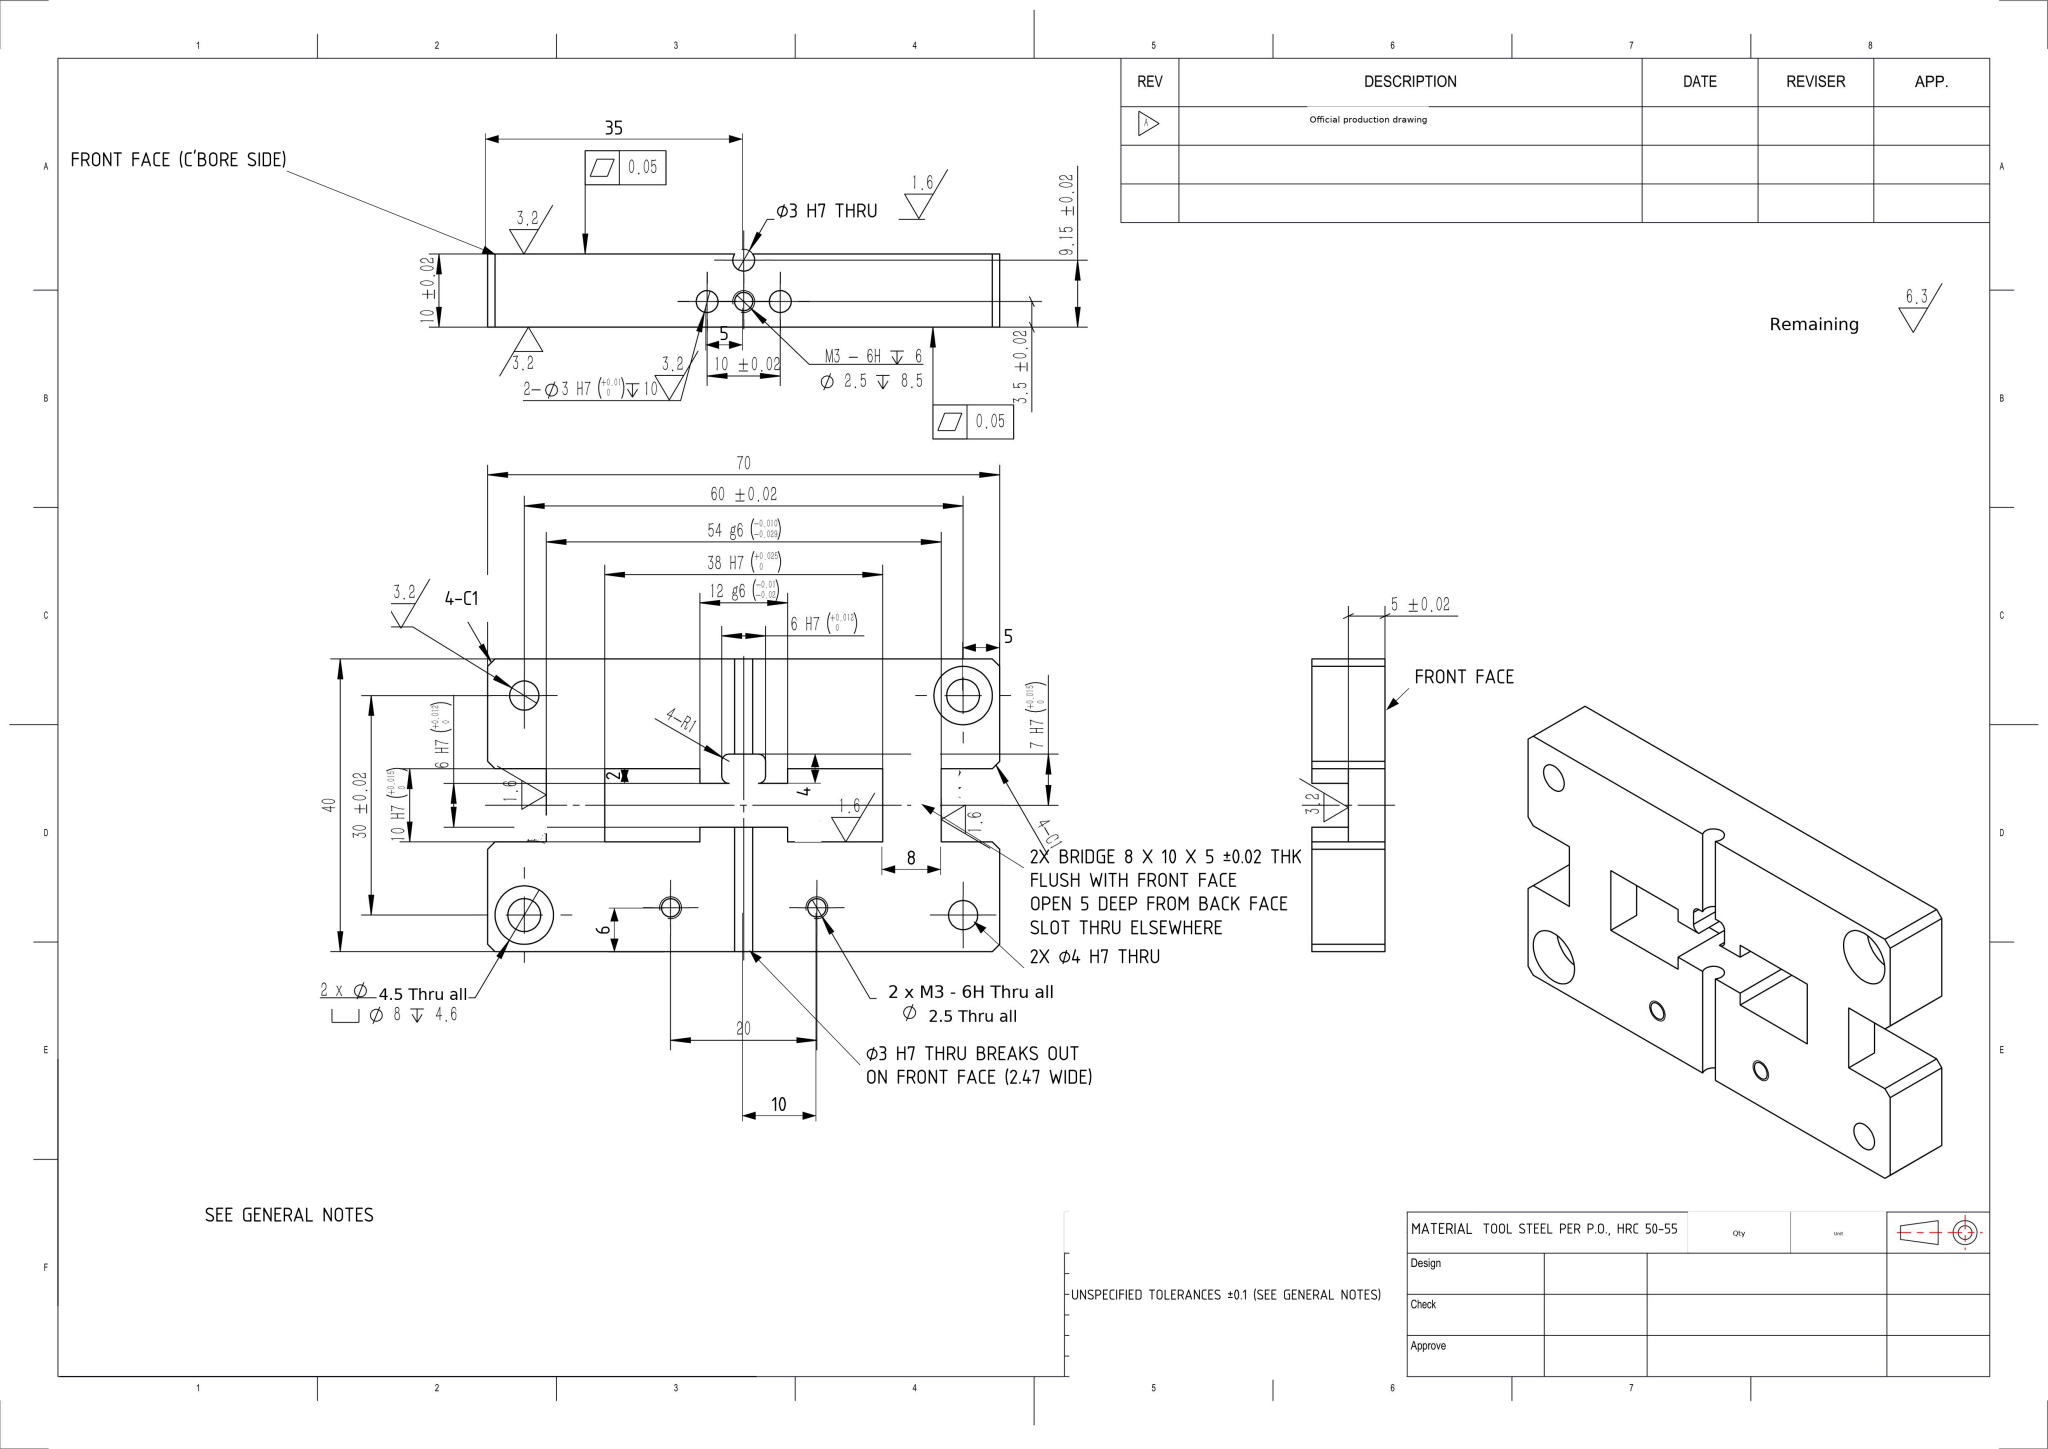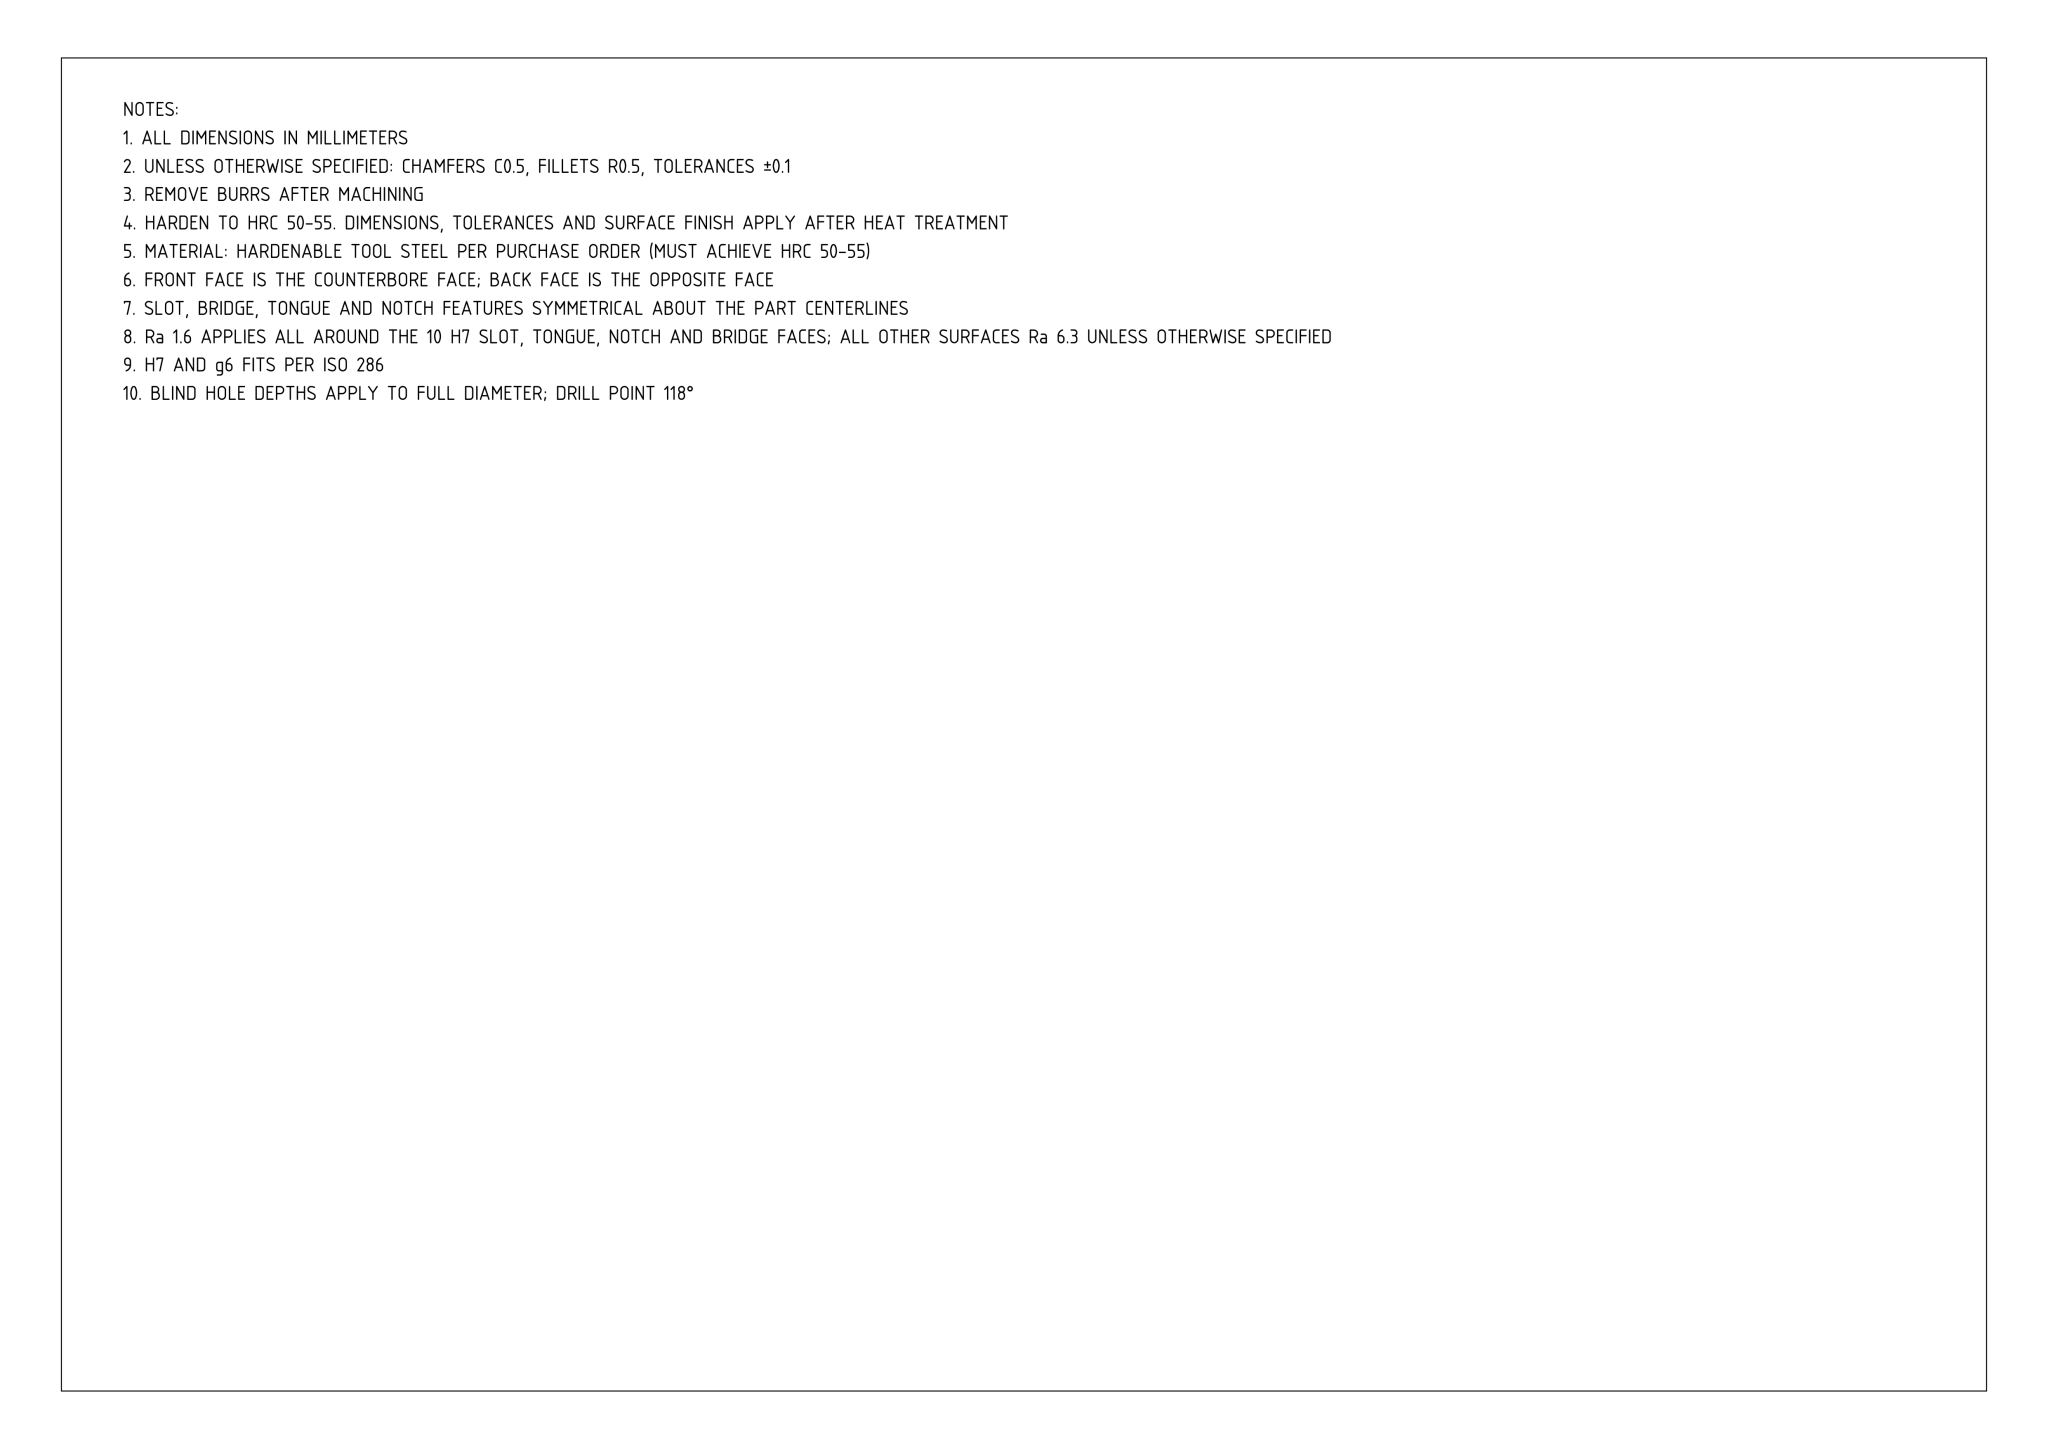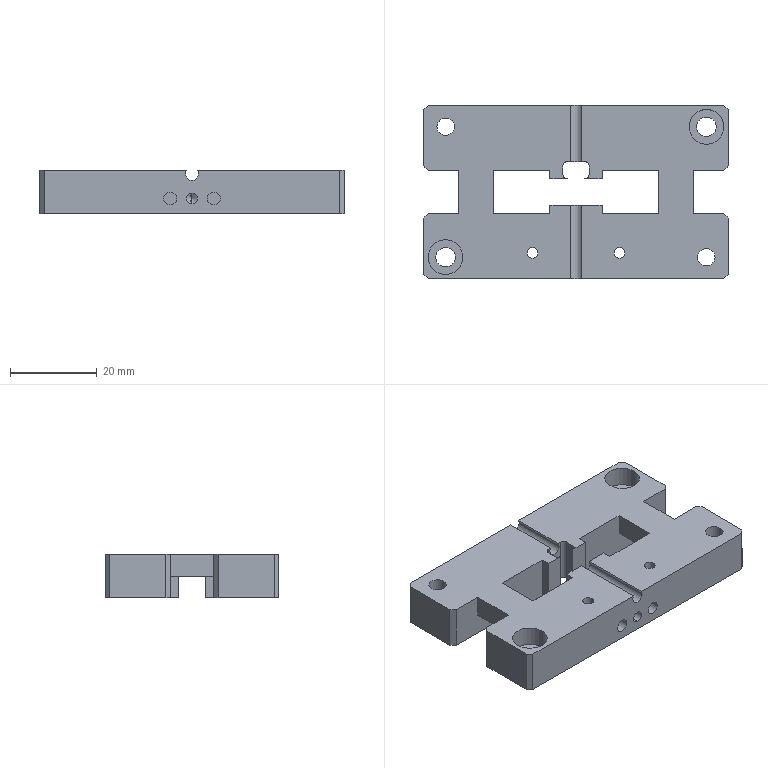Part | NX | mm | 1 solid | 76 faces | box 70 x 40 x 10 mm | volume 20662 mm3 | plane 42 | cylinder 32 | cone 2 | commonest cylinder face diameters 3 x10 2.5 x6 4 x4 8 x4 4.5 x4 2 x4